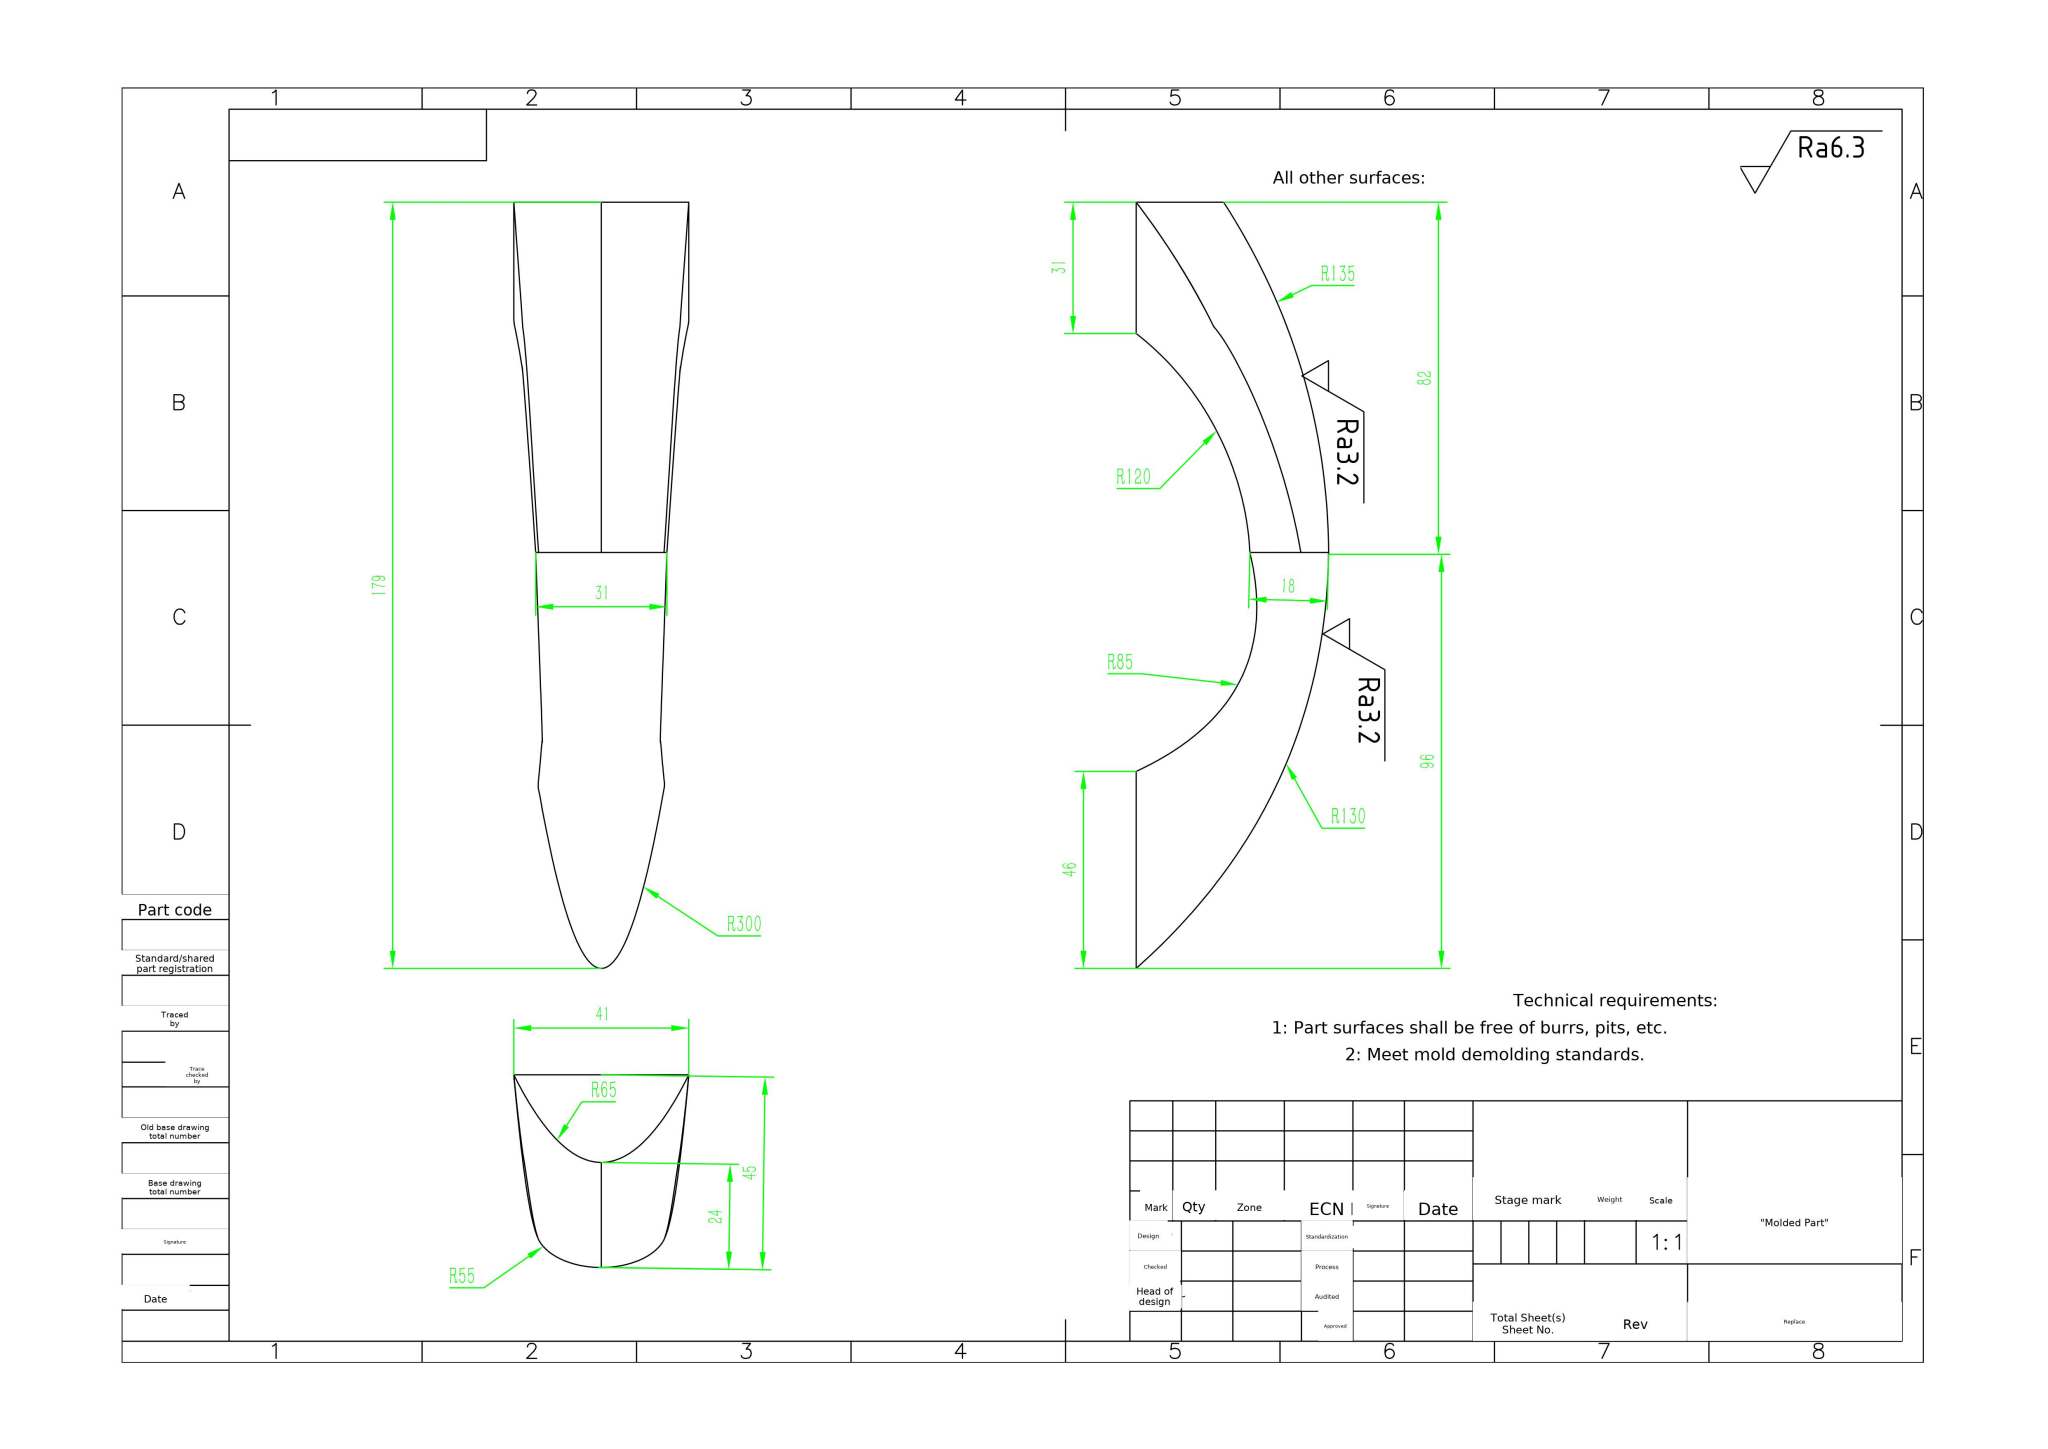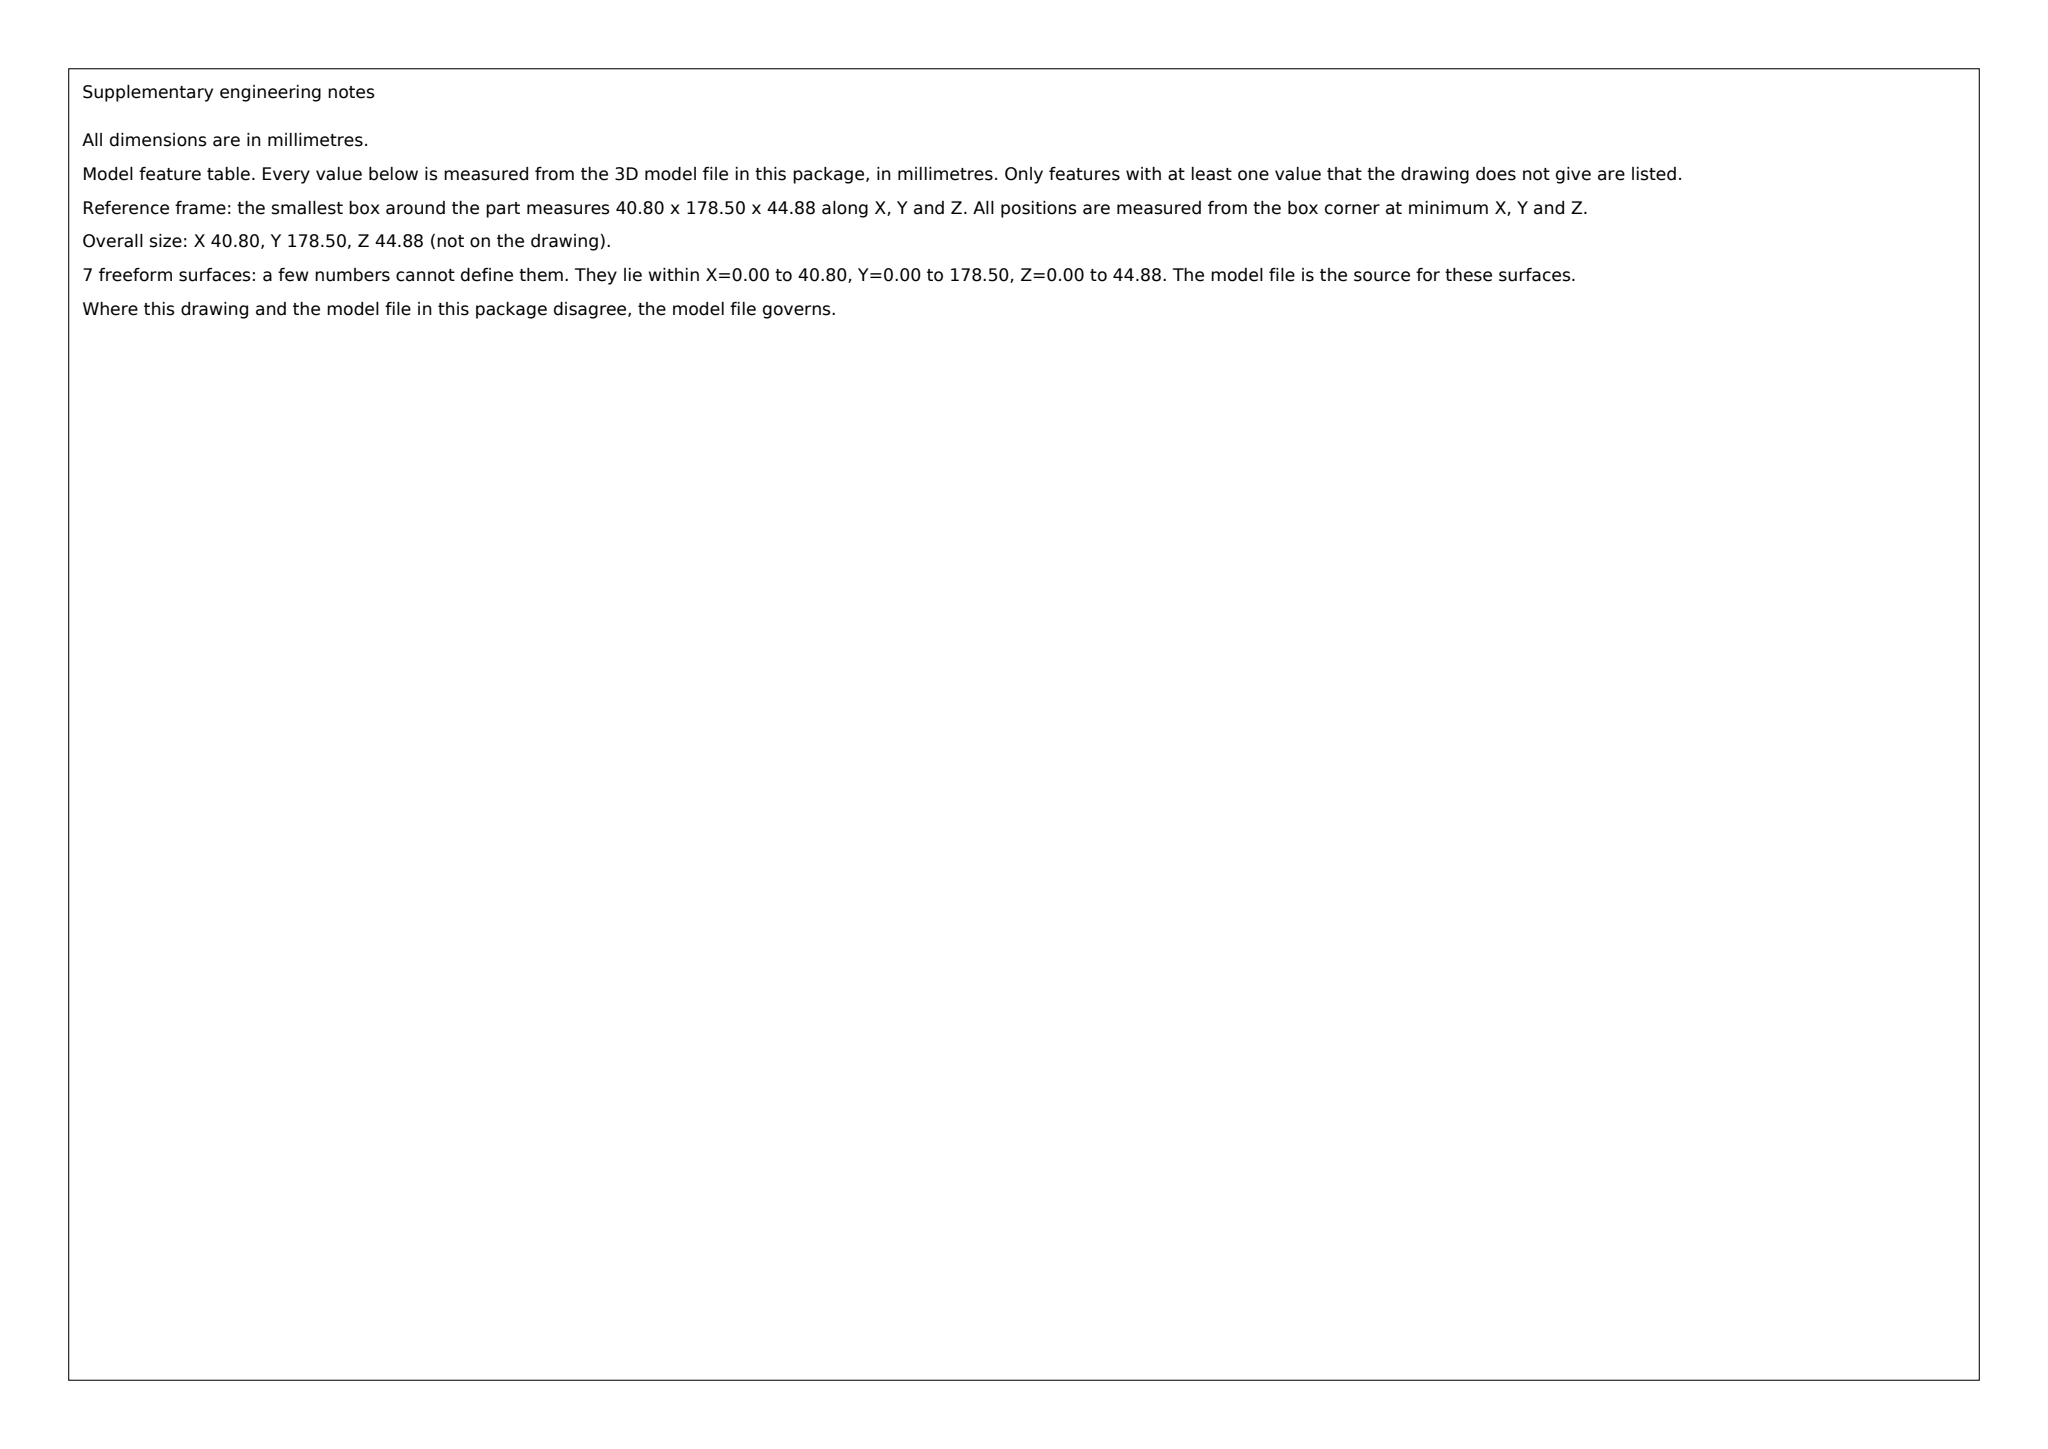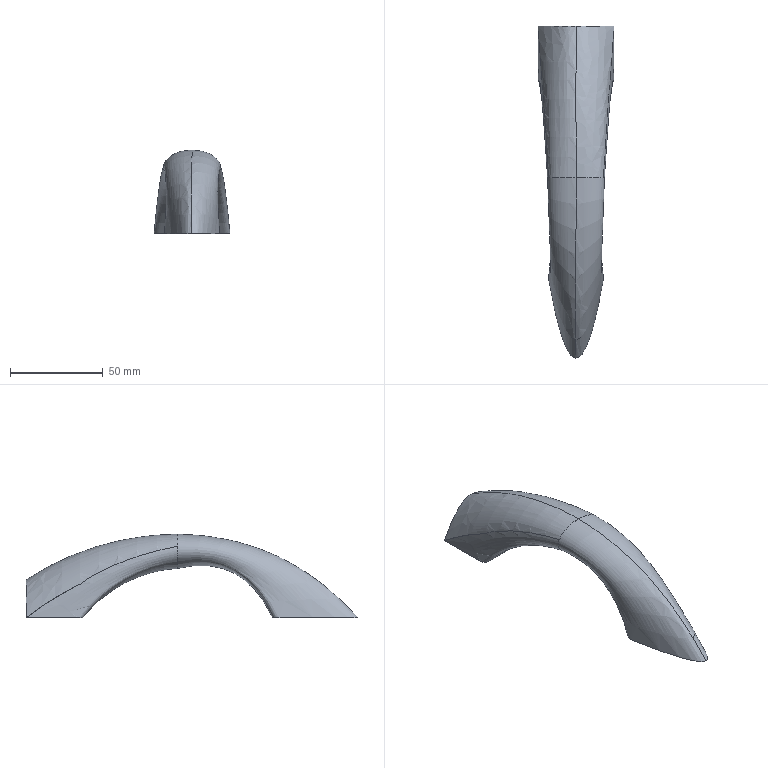Part | SolidWorks | mm | 1 solid | 10 faces | box 40.8 x 178.5 x 44.88 mm | volume 101811 mm3 | spline 7 | plane 3